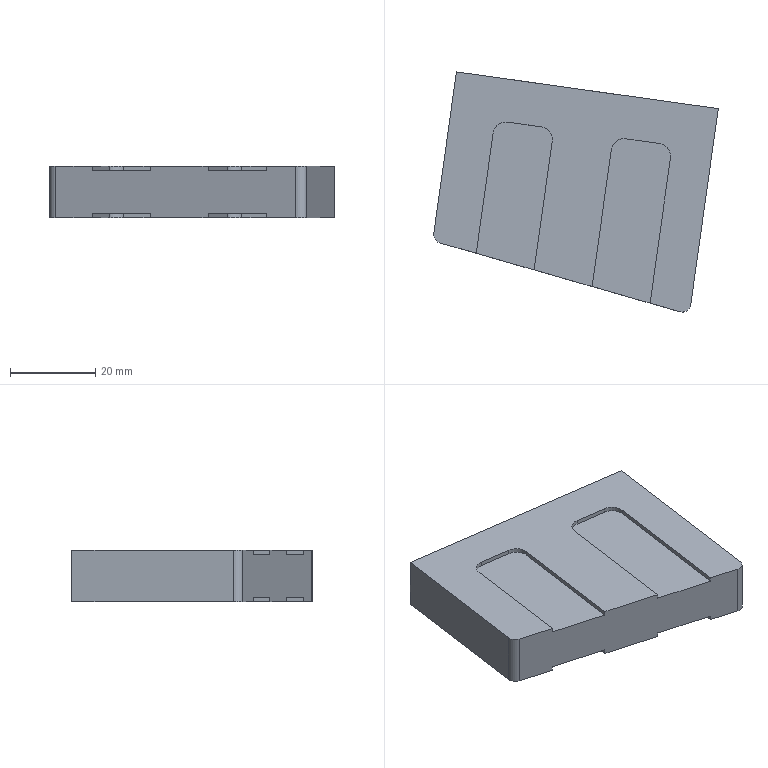Component | SolidWorks | Magazine-1 | 1 solid | 37 faces | box 66.74 x 56.31 x 12 mm | volume 14363 mm3 | plane 27 | cylinder 10 | commonest cylinder face diameters 6 x8 4 x2